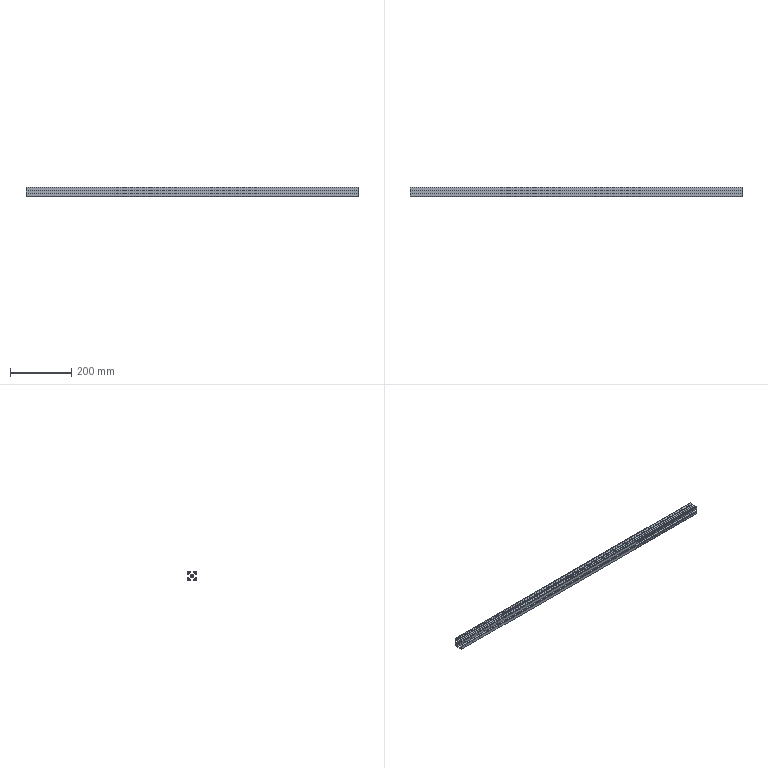Component | SolidWorks | 3030-1085-2 | 1 solid | 64 faces | box 1085 x 30 x 30 mm | volume 363092 mm3 | plane 46 | cylinder 18 | commonest cylinder face diameters 4.2 x8 0.6 x4 4 x4 6.8 x2
build123d program:
from build123d import *

# Parameters (mm, degrees)
SKETCH1_R           = 2.1
SKETCH1_R_2         = 3.4
BOSS_EXTRUDE1_DEPTH = 1085


with BuildPart() as part:
    # Sketch1 → Boss-Extrude1 (new body)
    with BuildSketch(Plane(origin=(0, 0, -100), x_dir=(-1, 0, 0), z_dir=(0, 0, -1))):
        with BuildLine():
            Line((15, 3.8), (15, 13.5))
            ThreePointArc((15, 13.5), (14.823, 14.323), (14.323, 15))
            Line((14.323, 15), (4, 15))
            Line((4, 15), (4, 13))
            Line((4, 13), (8.25, 13))
            Line((8.25, 13), (8.25, 9.664))
            Line((8.25, 9.664), (4.586, 6))
            Line((4.586, 6), (-4.586, 6))
            Line((-4.586, 6), (-8.25, 9.664))
            Line((-8.25, 9.664), (-8.25, 13))
            Line((-8.25, 13), (-4, 13))
            Line((-4, 13), (-4, 15))
            Line((-4, 15), (-14.323, 15))
            ThreePointArc((-14.323, 15), (-14.823, 14.323), (-15, 13.5))
            Line((-15, 13.5), (-15, 3.8))
            ThreePointArc((-15, 3.8), (-14.912, 3.588), (-14.7, 3.5))
            Line((-14.7, 3.5), (-13, 3.5))
            Line((-13, 3.5), (-13, 8.25))
            Line((-13, 8.25), (-9.664, 8.25))
            Line((-9.664, 8.25), (-6, 4.586))
            Line((-6, 4.586), (-6, -4.586))
            Line((-6, -4.586), (-9.664, -8.25))
            Line((-9.664, -8.25), (-13, -8.25))
            Line((-13, -8.25), (-13, -4.5))
            Line((-13, -4.5), (-14.7, -4.5))
            ThreePointArc((-14.7, -4.5), (-14.912, -4.588), (-15, -4.8))
            Line((-15, -4.8), (-15, -13.5))
            ThreePointArc((-15, -13.5), (-14.823, -14.323), (-14.323, -15))
            Line((-14.323, -15), (-4, -15))
            Line((-4, -15), (-4, -13))
            Line((-4, -13), (-8.25, -13))
            Line((-8.25, -13), (-8.25, -9.664))
            Line((-8.25, -9.664), (-4.586, -6))
            Line((-4.586, -6), (4.586, -6))
            Line((4.586, -6), (8.25, -9.664))
            Line((8.25, -9.664), (8.25, -13))
            Line((8.25, -13), (4, -13))
            Line((4, -13), (4, -15))
            Line((4, -15), (14.323, -15))
            ThreePointArc((14.323, -15), (14.823, -14.323), (15, -13.5))
            Line((15, -13.5), (15, -4.8))
            ThreePointArc((15, -4.8), (14.912, -4.588), (14.7, -4.5))
            Line((14.7, -4.5), (13, -4.5))
            Line((13, -4.5), (13, -8.25))
            Line((13, -8.25), (9.664, -8.25))
            Line((9.664, -8.25), (6, -4.586))
            Line((6, -4.586), (6, 4.586))
            Line((6, 4.586), (9.664, 8.25))
            Line((9.664, 8.25), (13, 8.25))
            Line((13, 8.25), (13, 3.5))
            Line((13, 3.5), (14.7, 3.5))
            ThreePointArc((14.7, 3.5), (14.912, 3.588), (15, 3.8))
        make_face()
        with Locations(Location((11.625, 11.625, 0), (0, 0, 180))):
            Circle(SKETCH1_R, mode=Mode.SUBTRACT)
        with Locations(Location((11.625, -11.625, 0), (0, 0, 180))):
            Circle(SKETCH1_R, mode=Mode.SUBTRACT)
        with Locations(Location((0, 0, 0), (0, 0, 180))):
            Circle(SKETCH1_R_2, mode=Mode.SUBTRACT)
        with Locations(Location((-11.625, 11.625, 0), (0, 0, 180))):
            Circle(SKETCH1_R, mode=Mode.SUBTRACT)
        with Locations(Location((-11.625, -11.625, 0), (0, 0, 180))):
            Circle(SKETCH1_R, mode=Mode.SUBTRACT)
    extrude(amount=-BOSS_EXTRUDE1_DEPTH)


solid = part.part

# Placed as in the assembly
solid = solid.moved(Location((101.953, 637.523, -435), (0, 90, 0)))